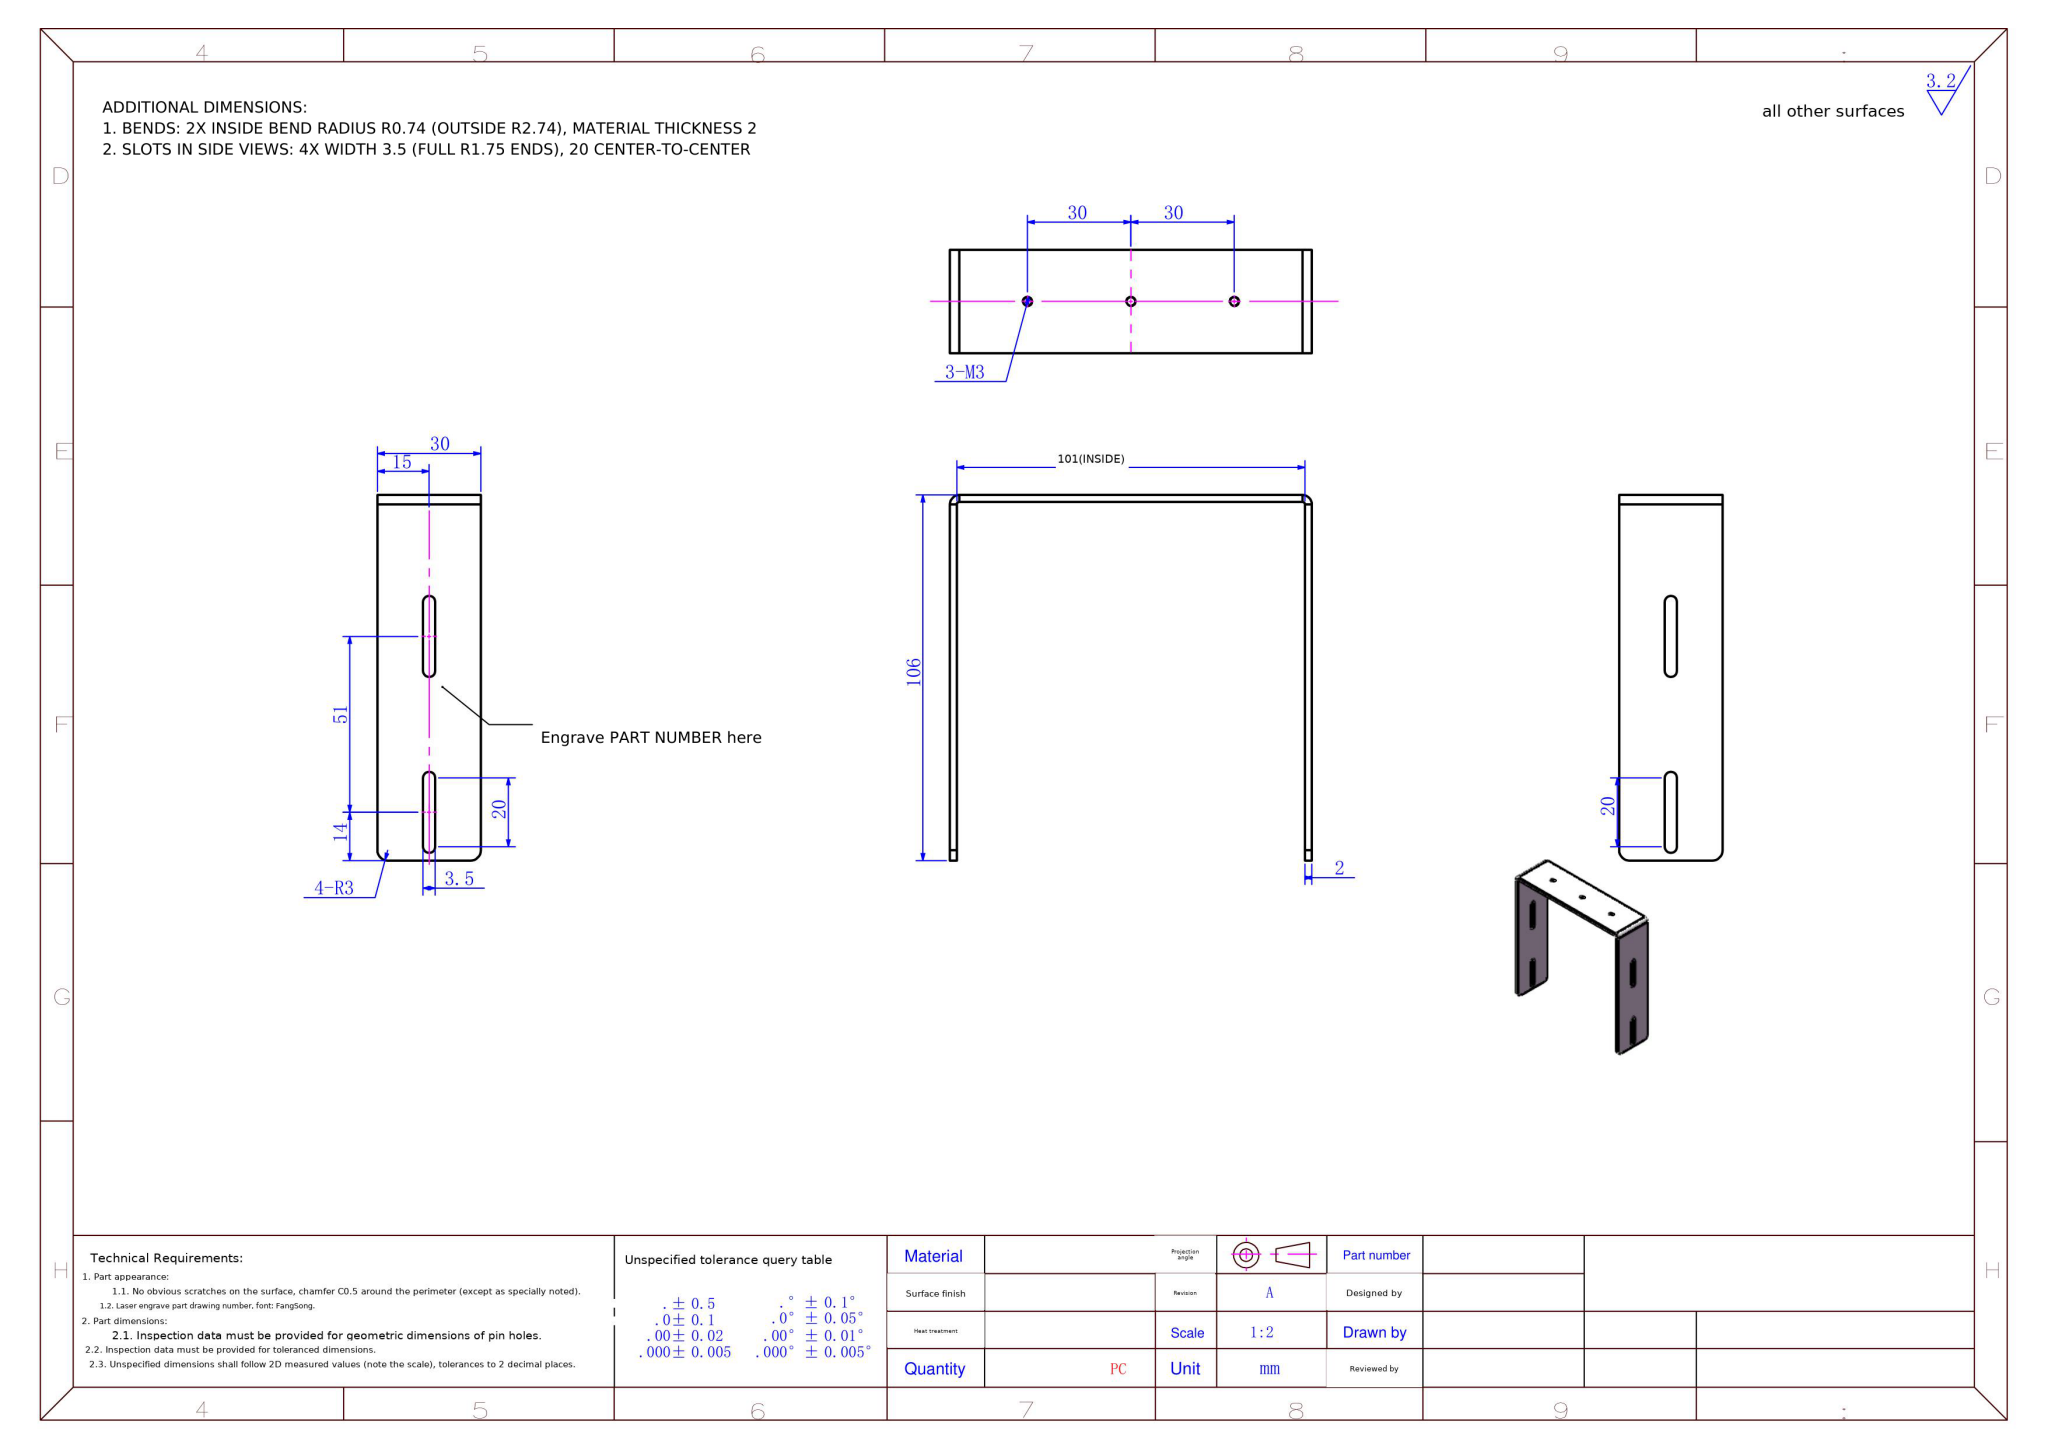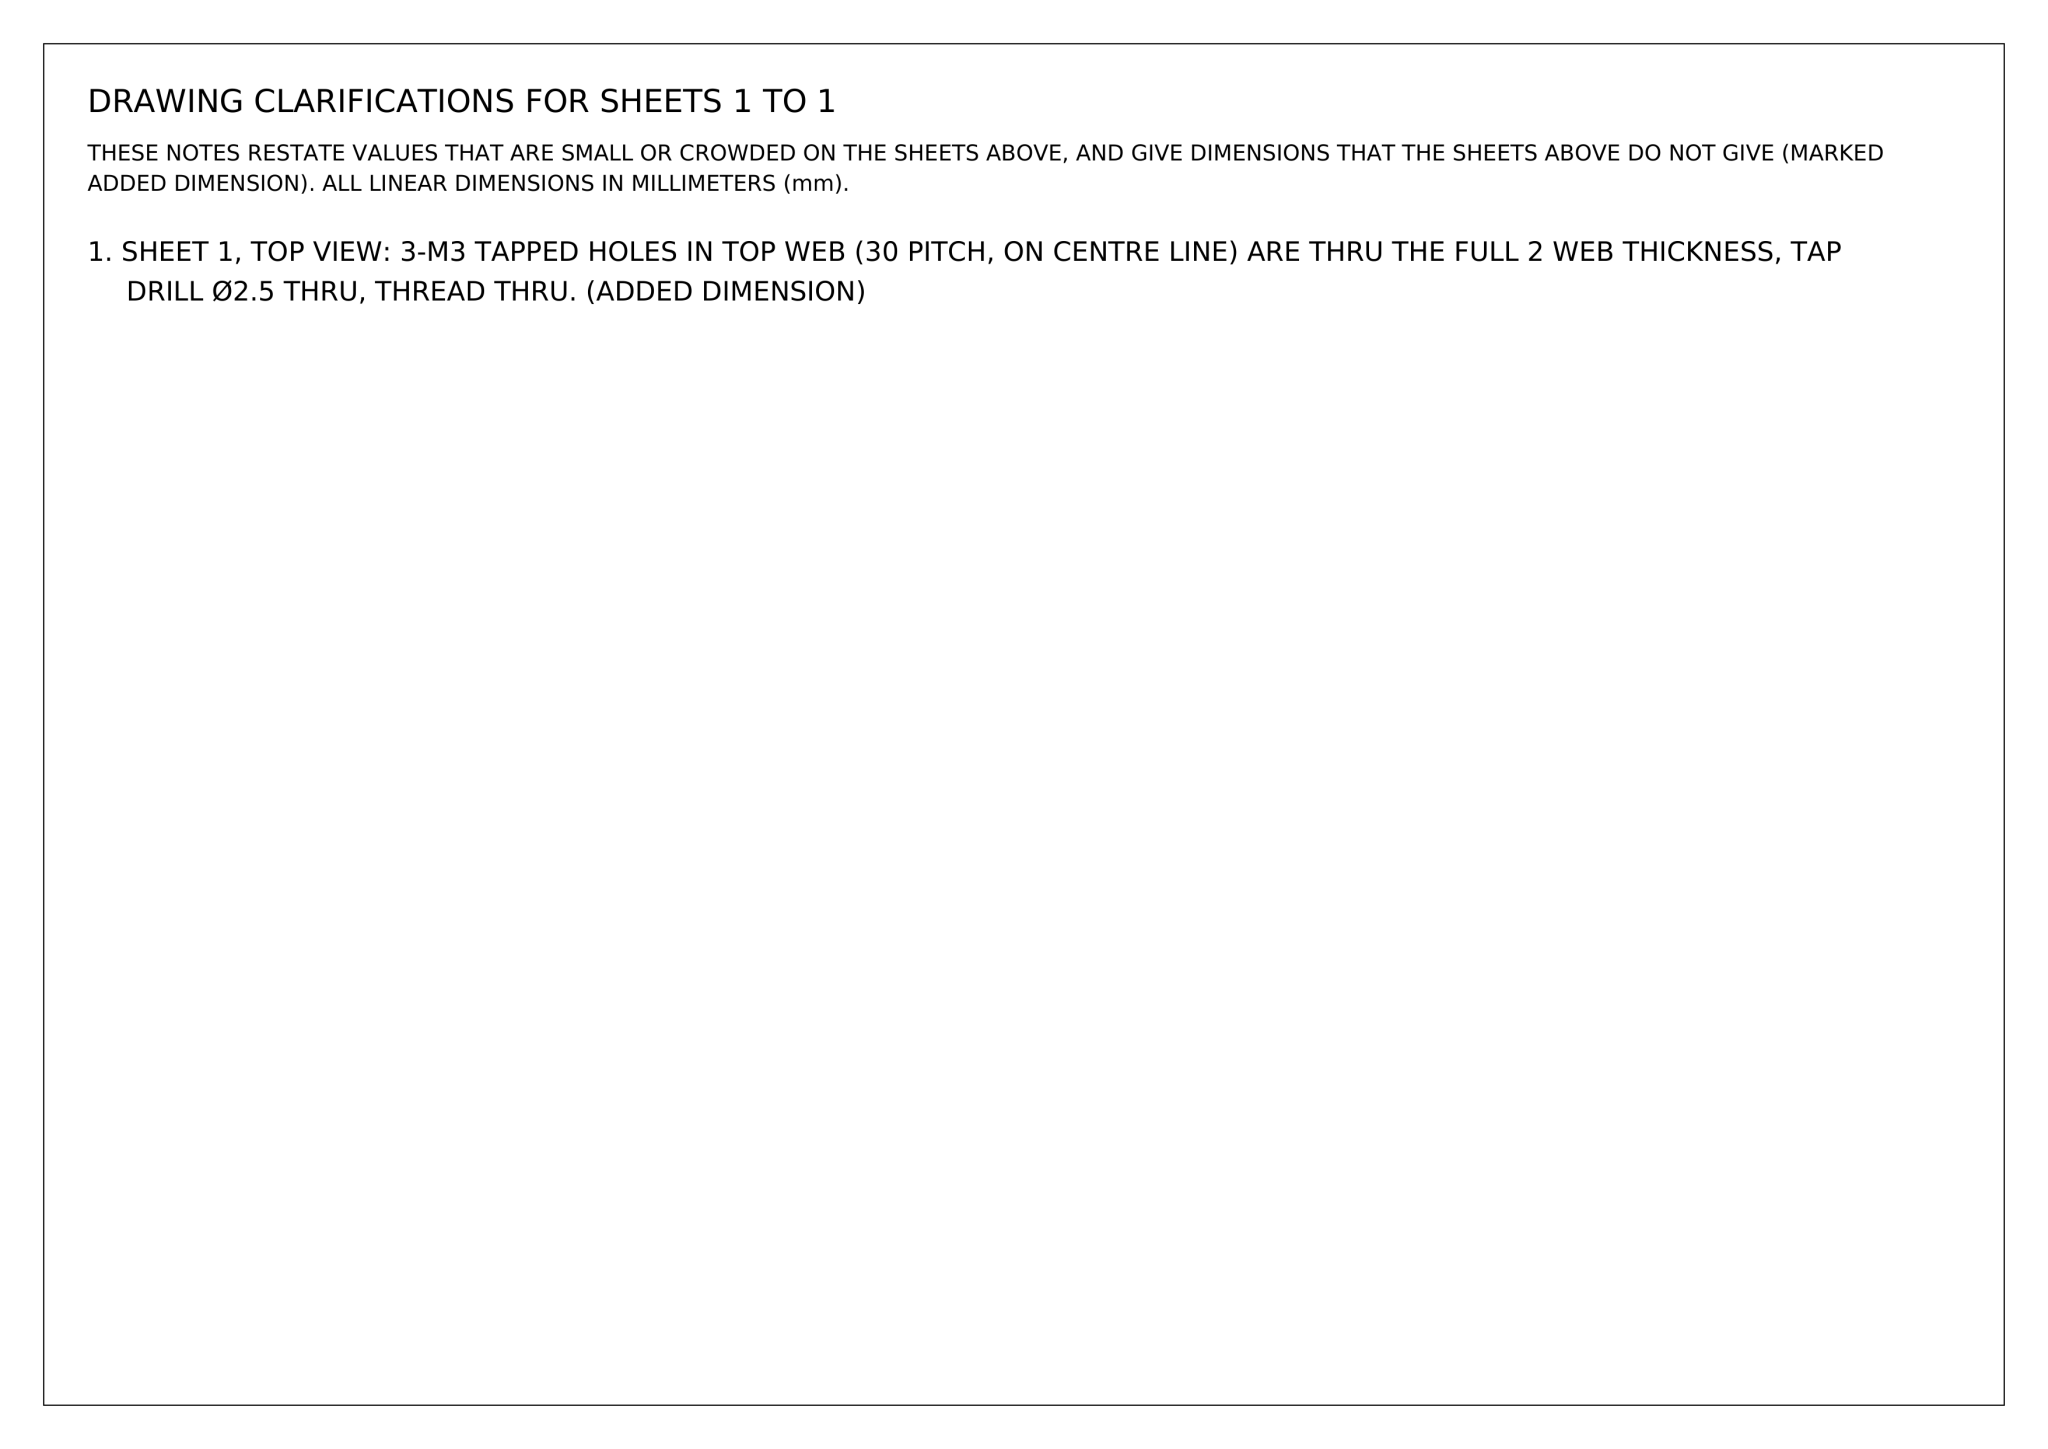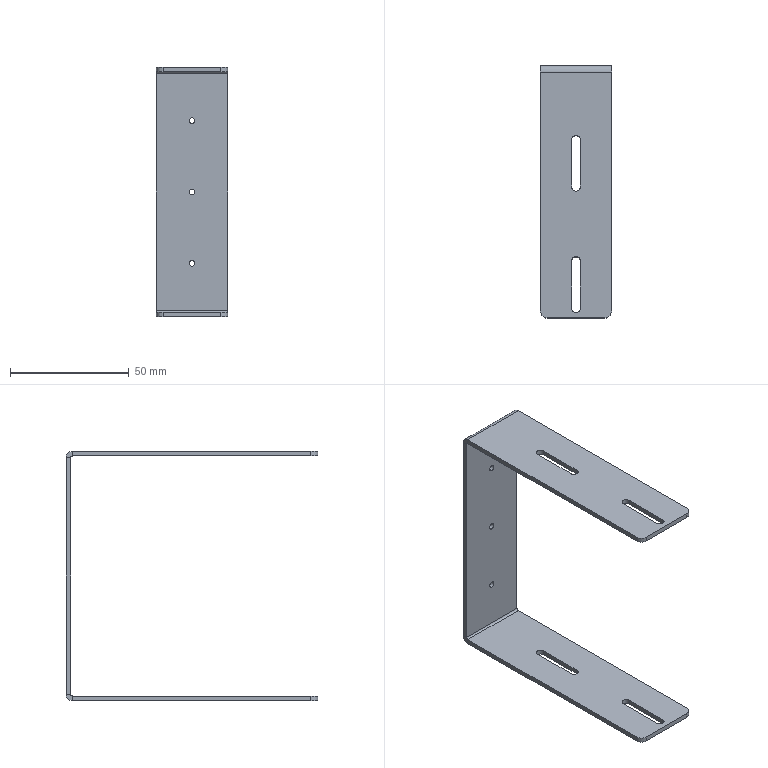Part | NX | mm | 1 solid | 48 faces | box 30 x 106 x 105 mm | volume 18009 mm3 | plane 26 | cylinder 22 | commonest cylinder face diameters 3.5 x8 2.5 x6 6 x4 1.473 x2 5.473 x2